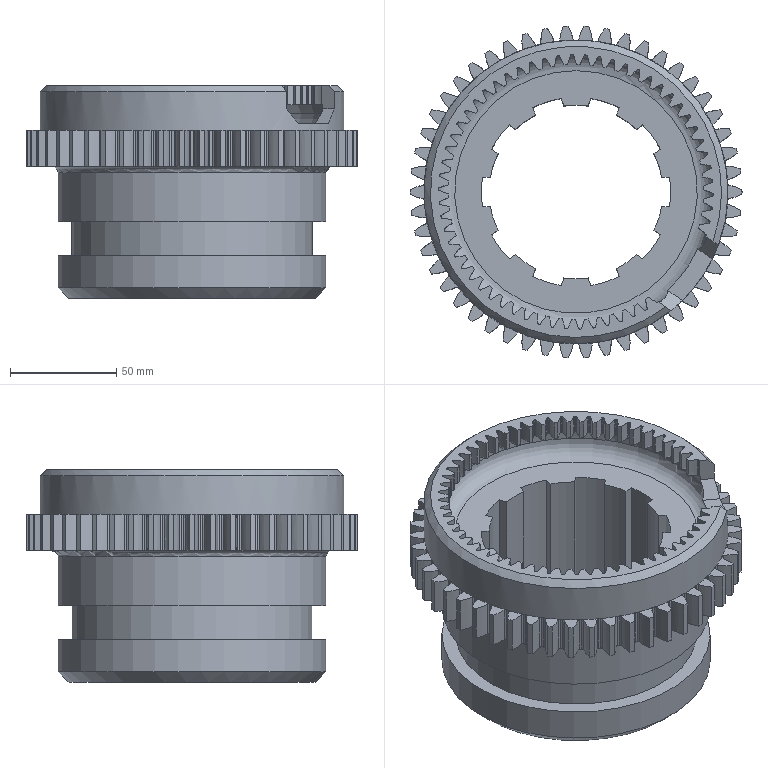Component | NX | CA6140-ZHUZHOU-CHILUN2 | 1 solid | 800 faces | volume 640725 mm3 | other 476 | cylinder 188 | plane 132 | torus 2 | cone 2 | commonest cylinder face diameters 129 x57 120 x56 142.5 x50 81.64 x10 89 x10 126 x2 142.8 x1 130 x1